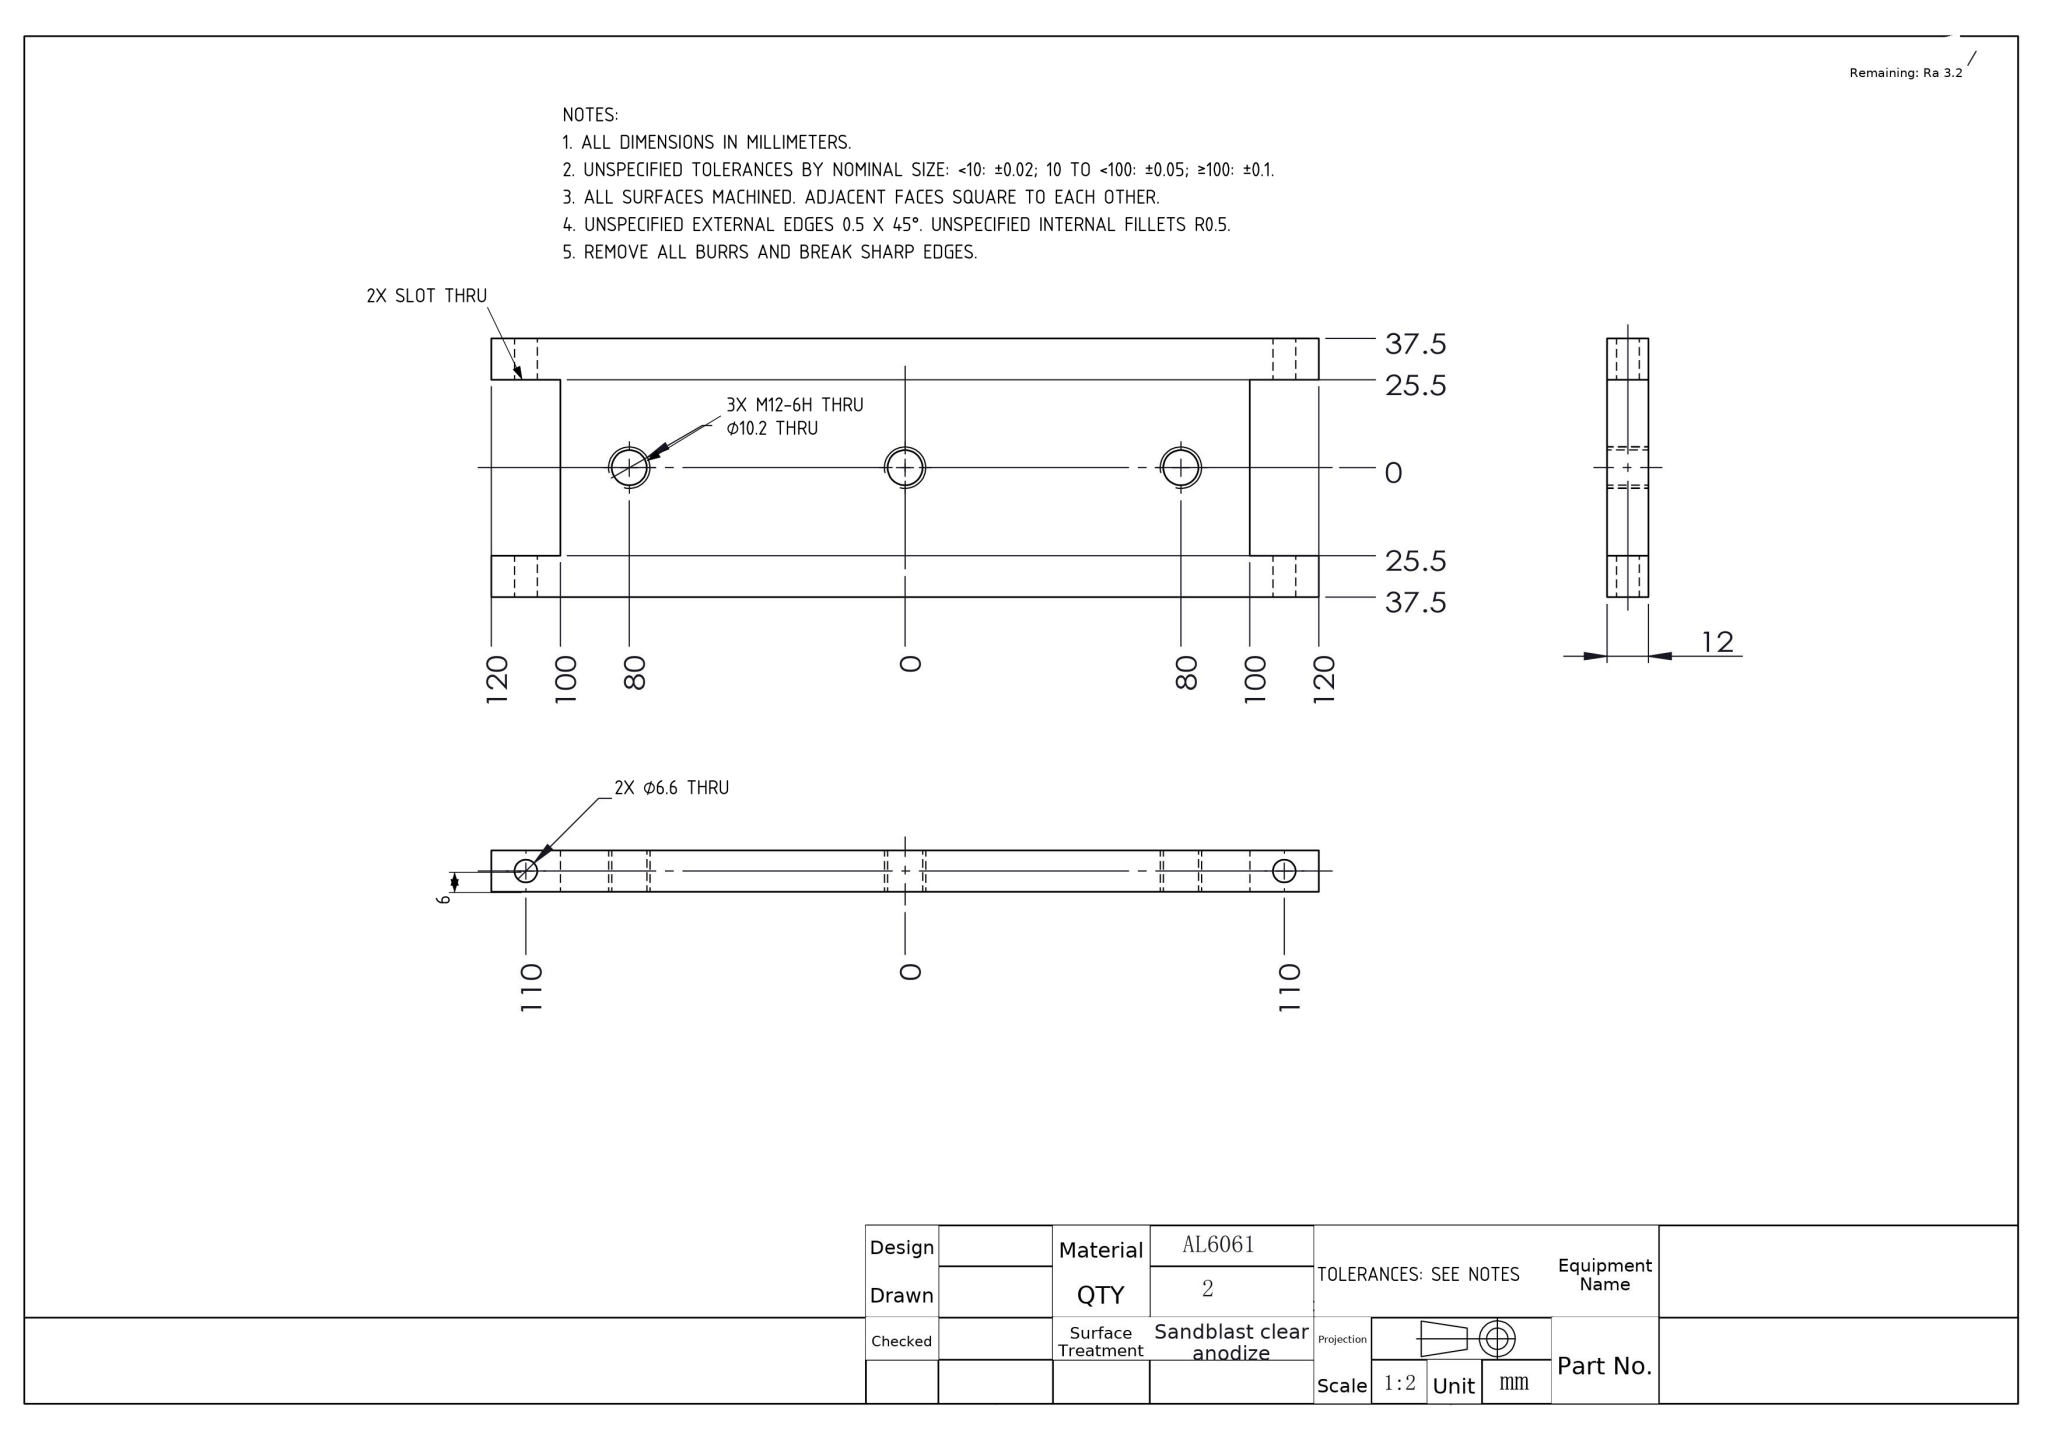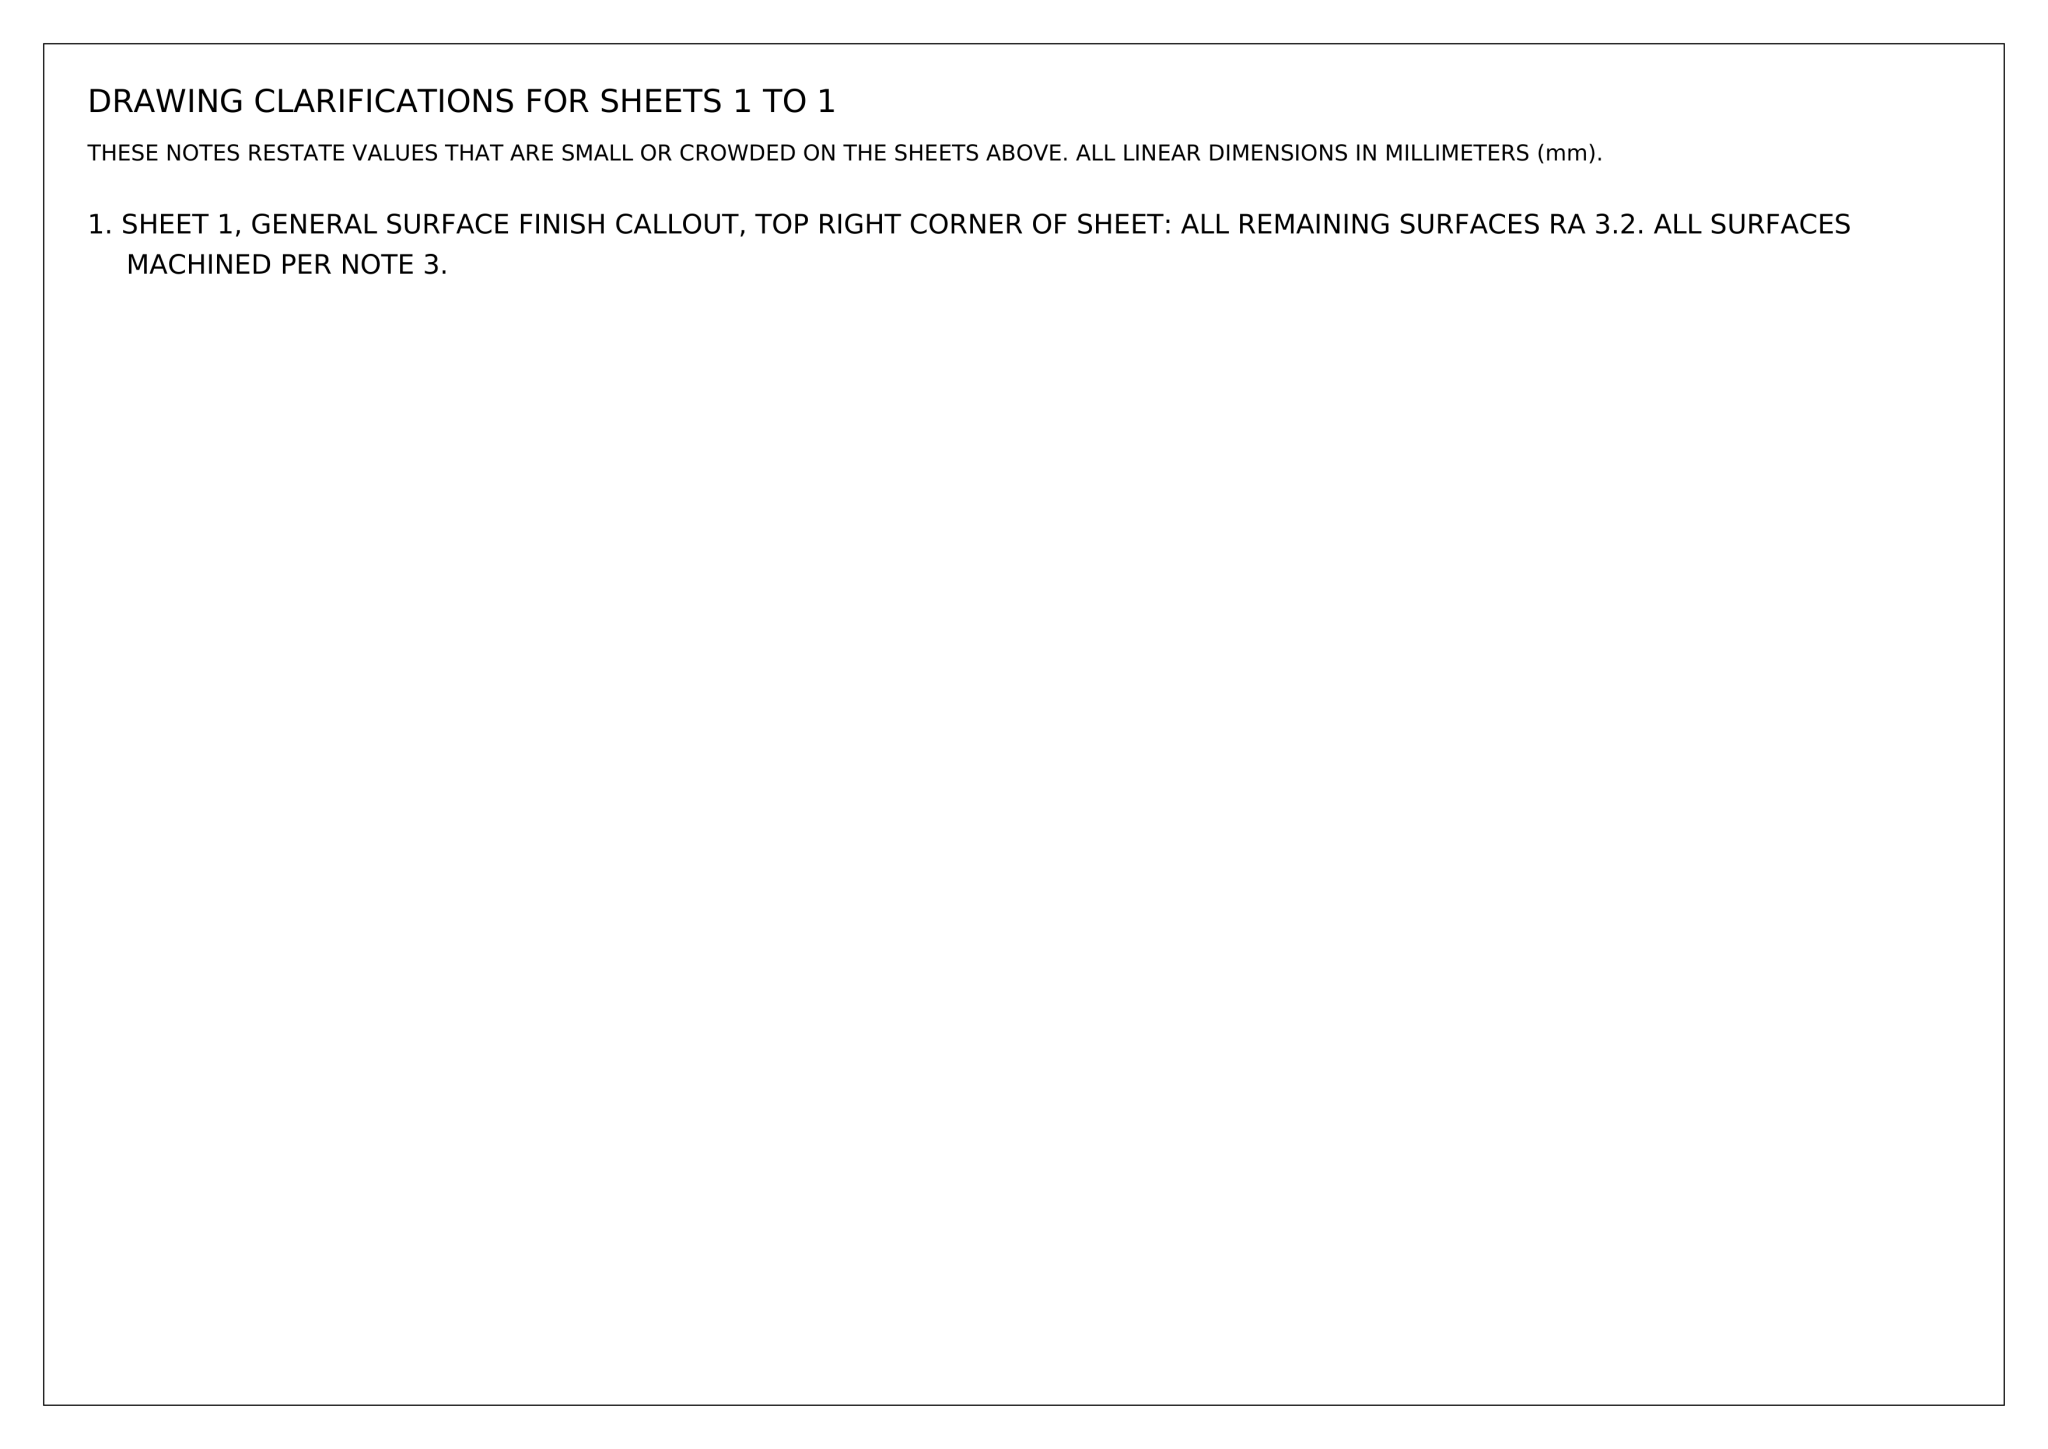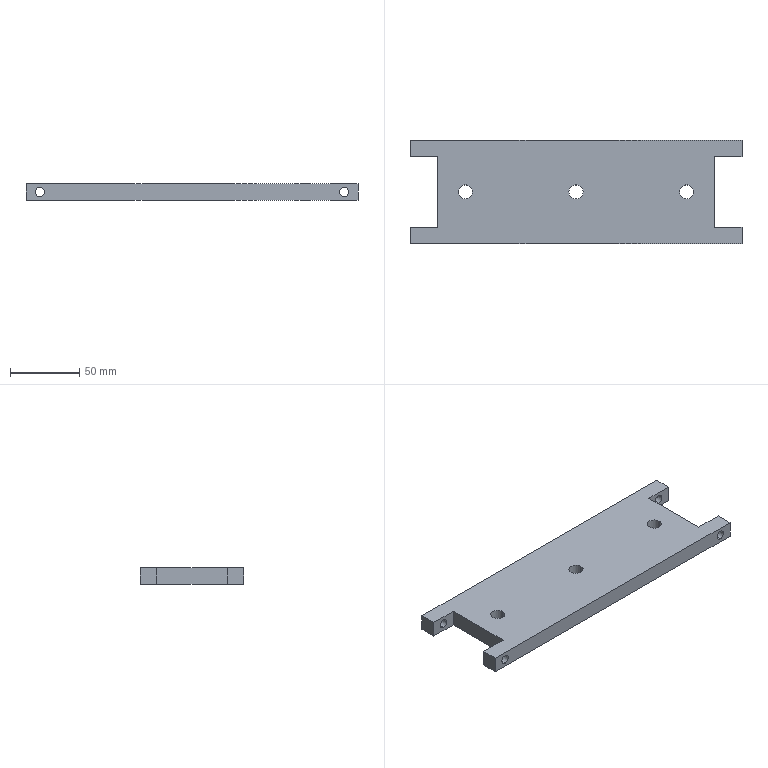Part | NX | mm | 1 solid | 28 faces | box 240 x 75 x 12 mm | volume 186936 mm3 | cylinder 14 | plane 14 | commonest cylinder face diameters 6.6 x8 10.2 x6